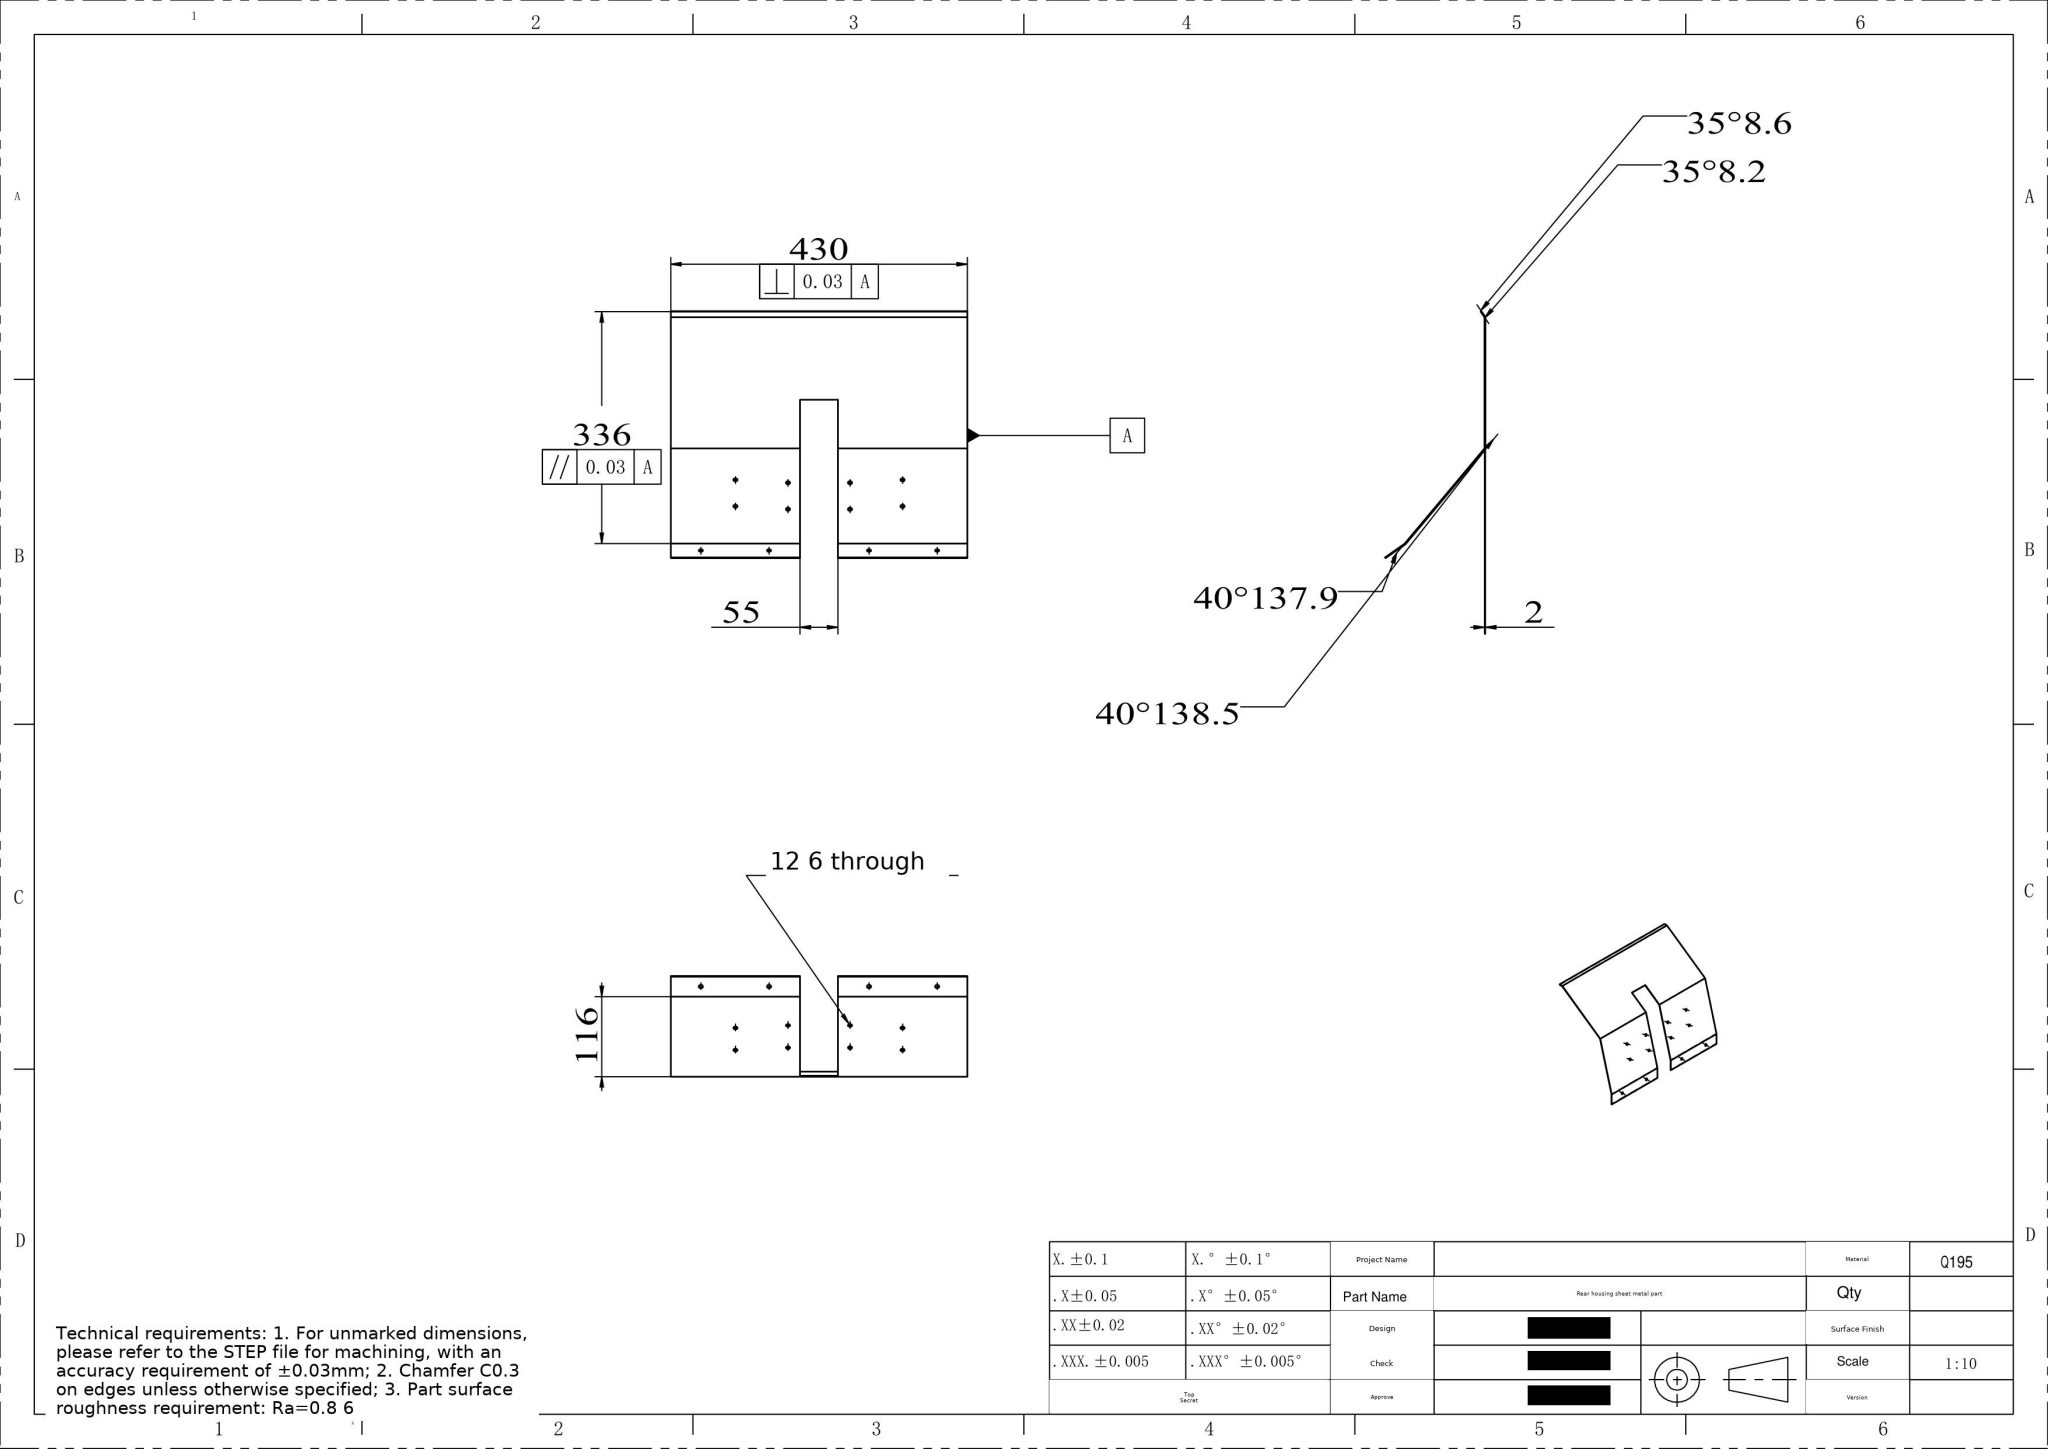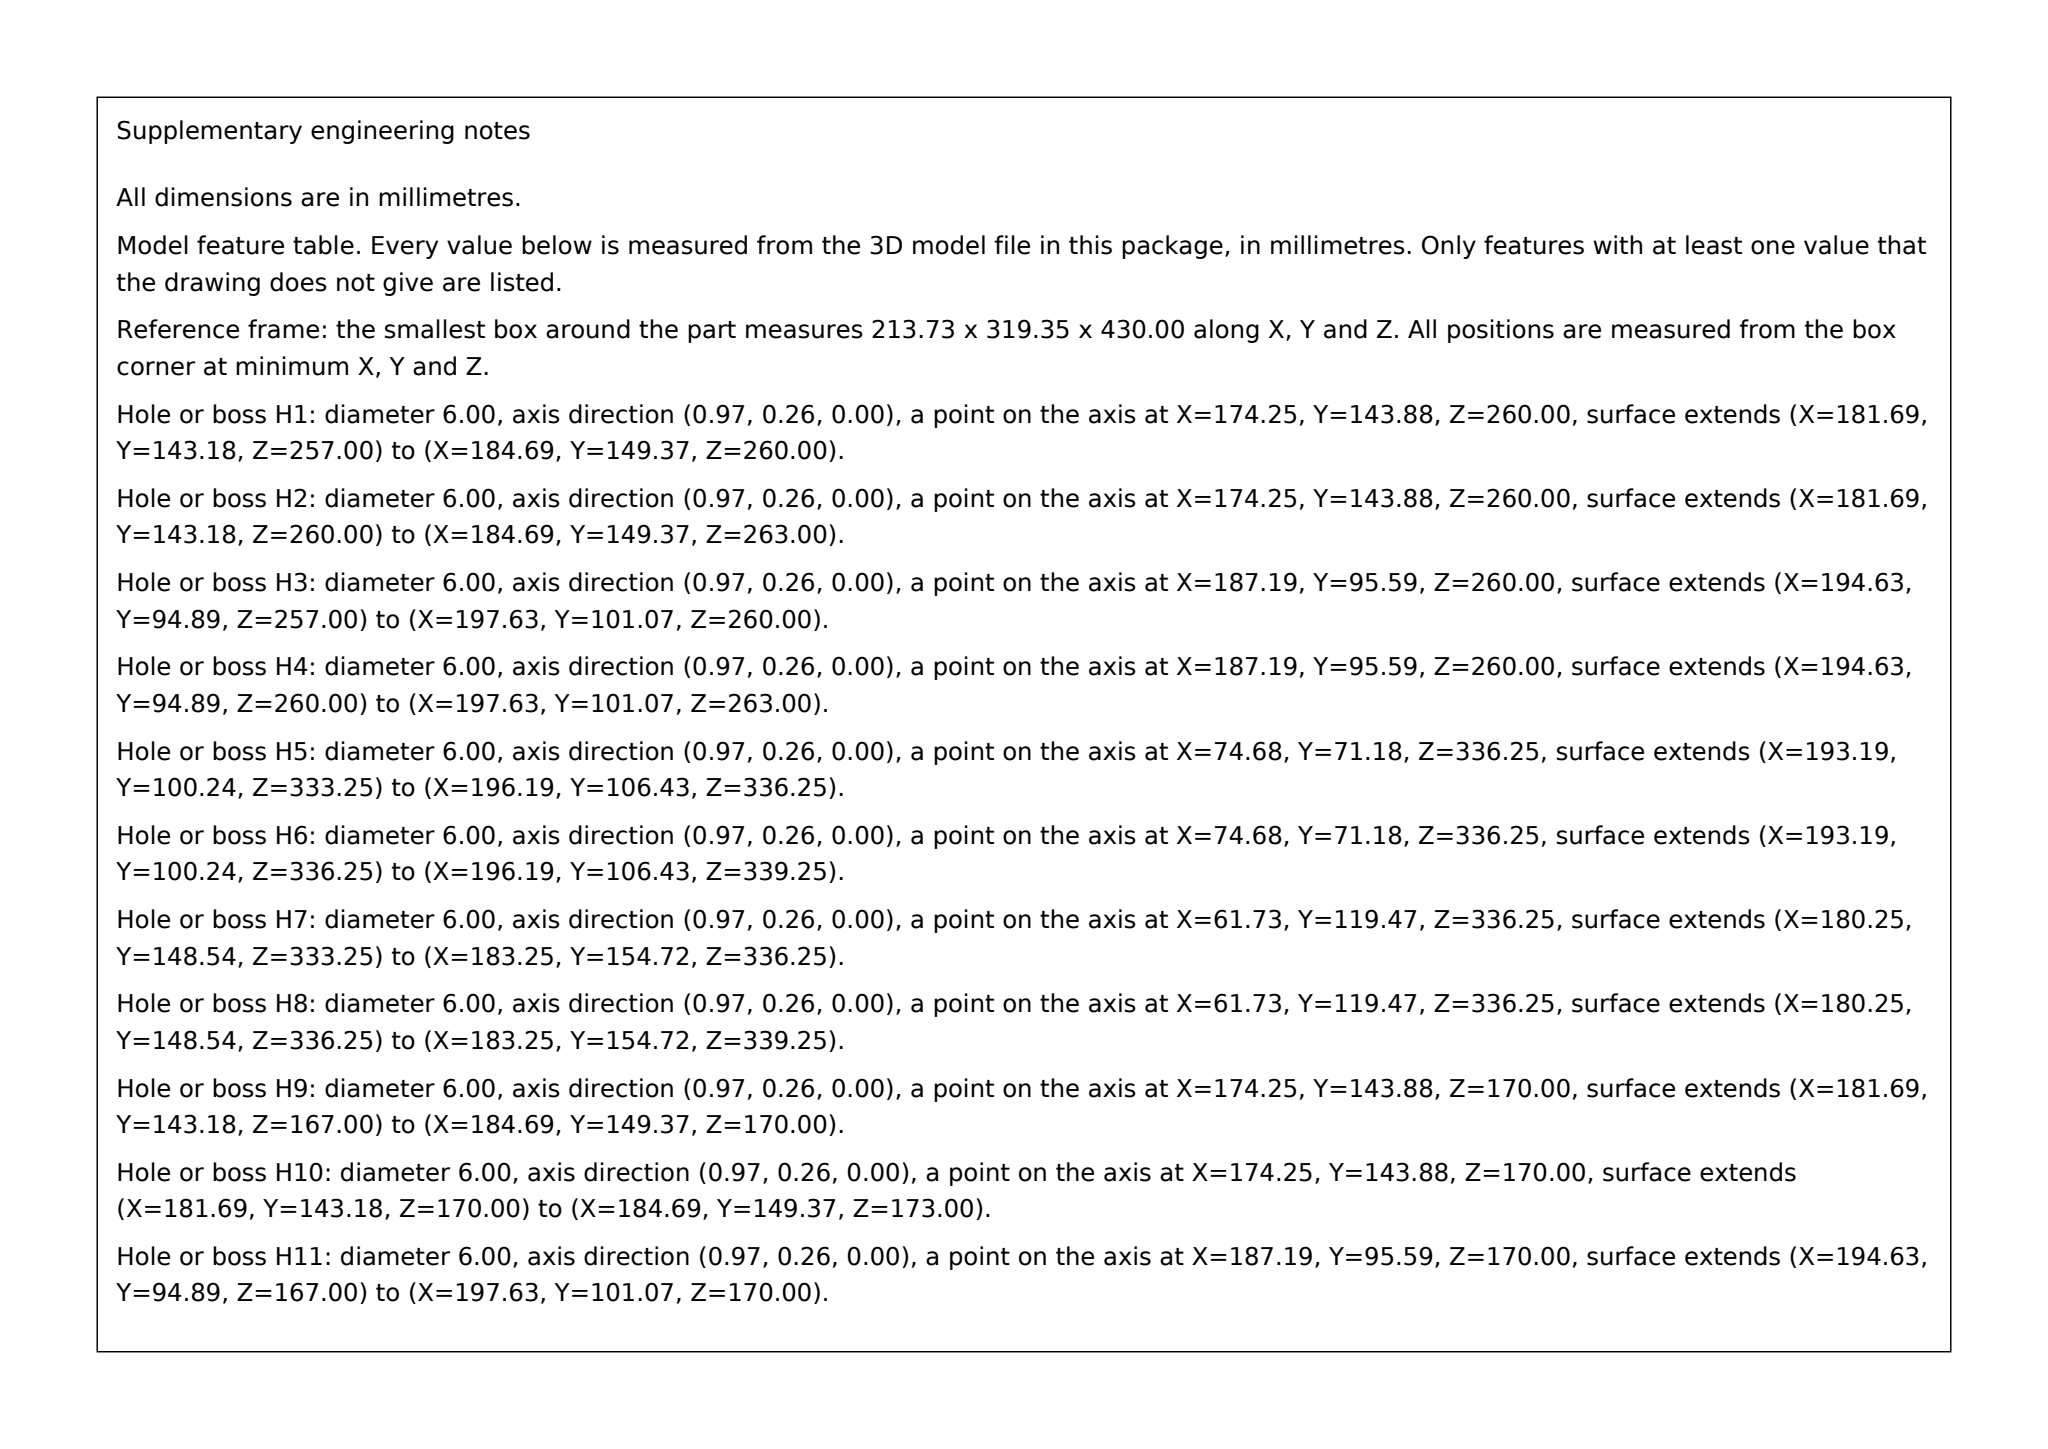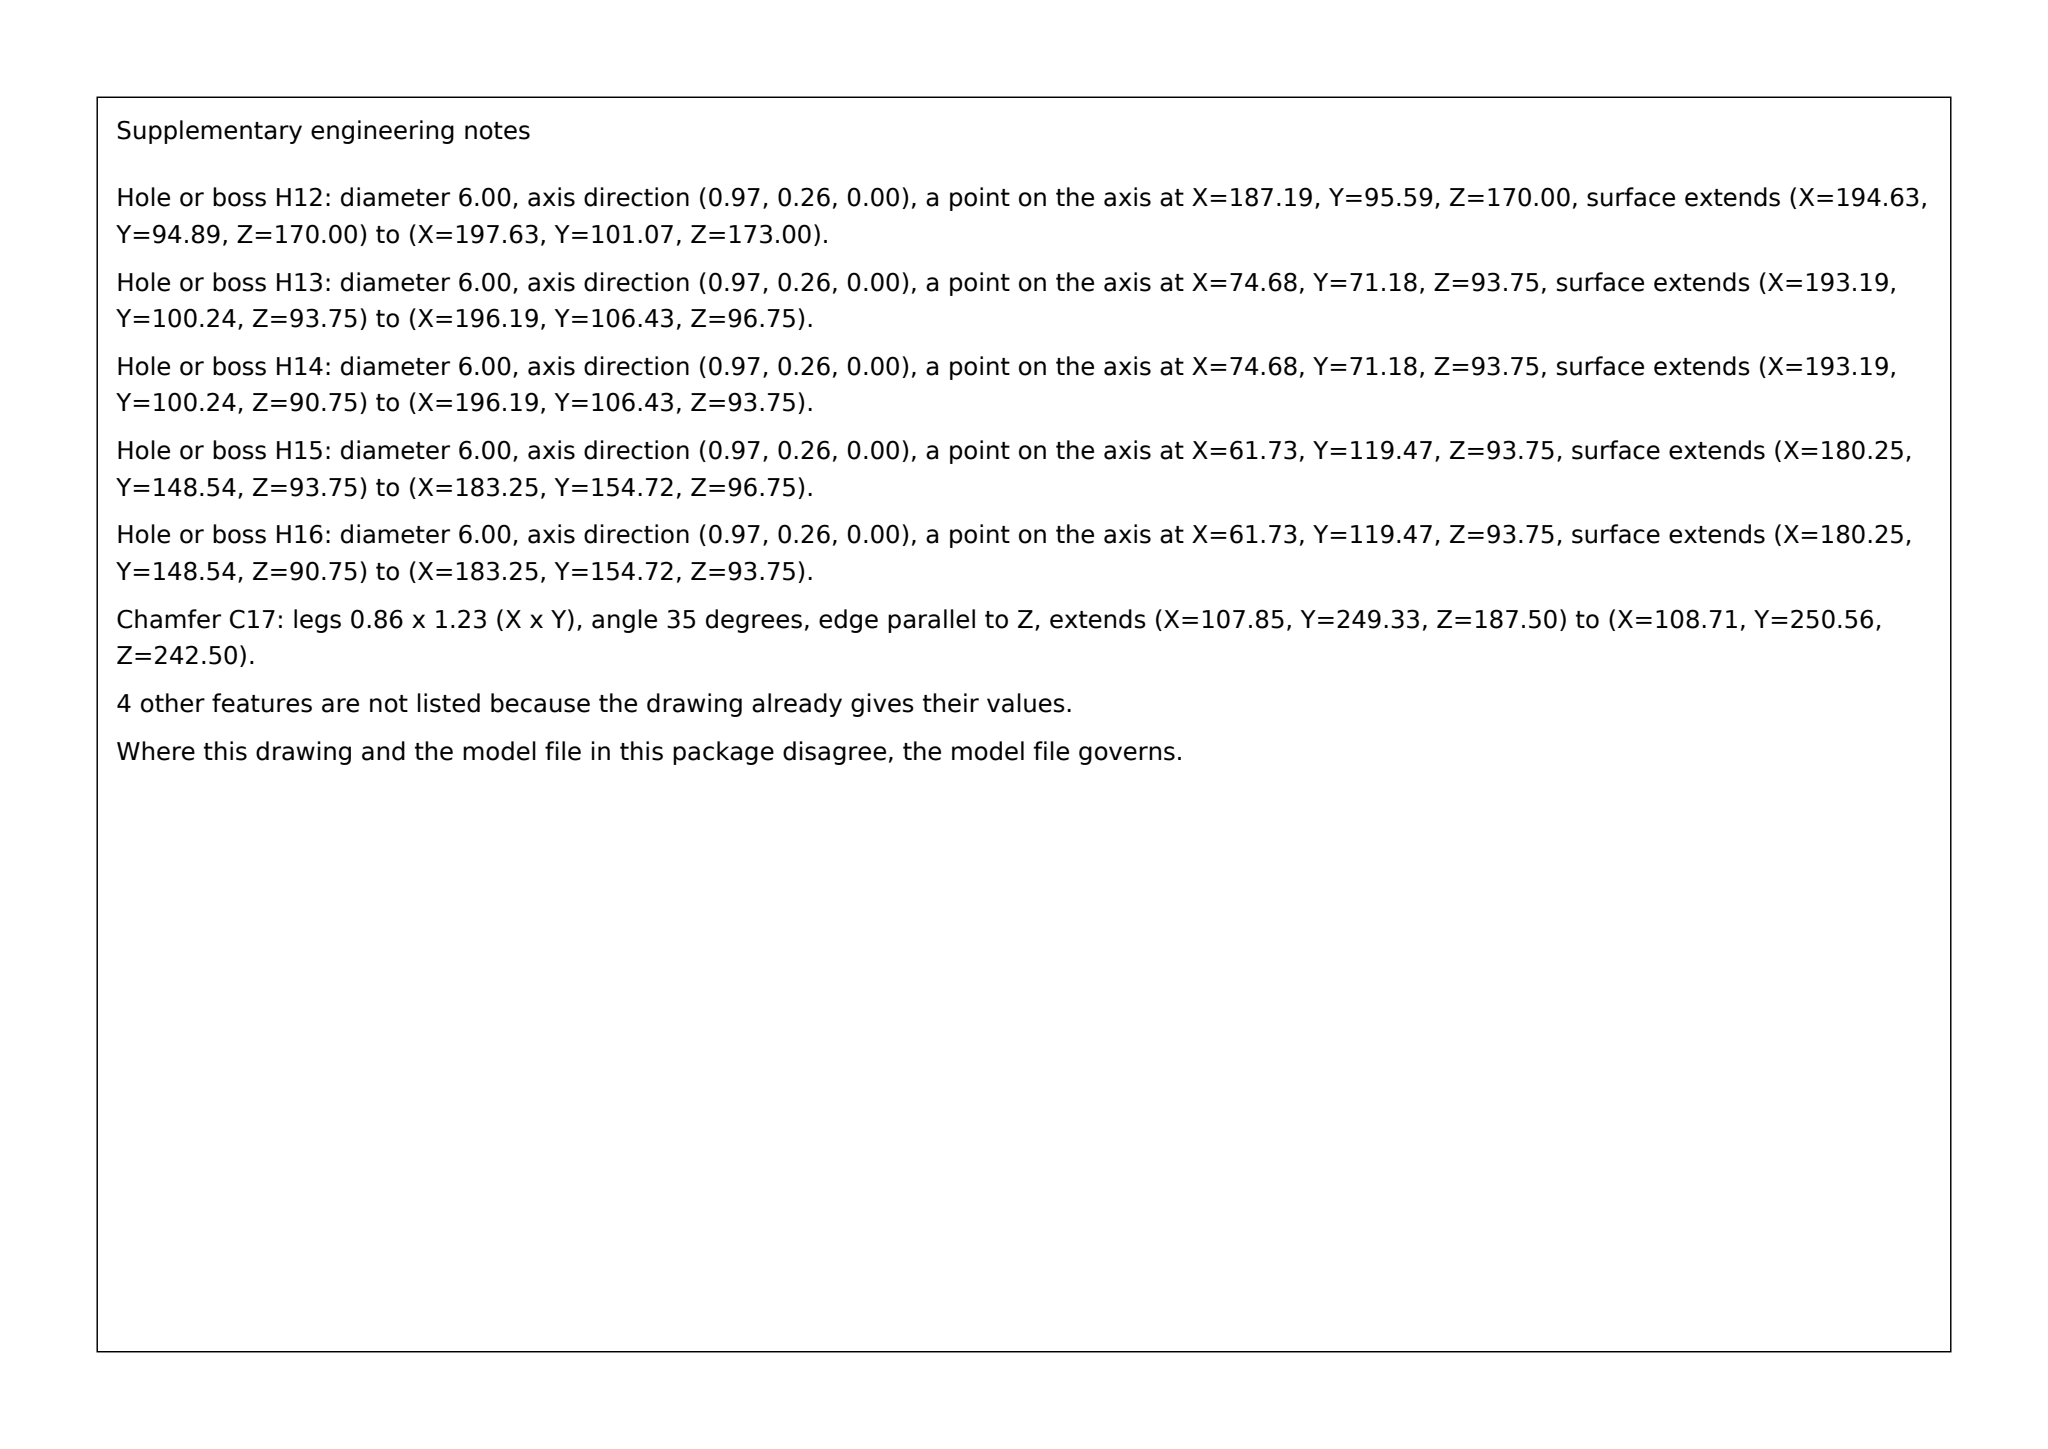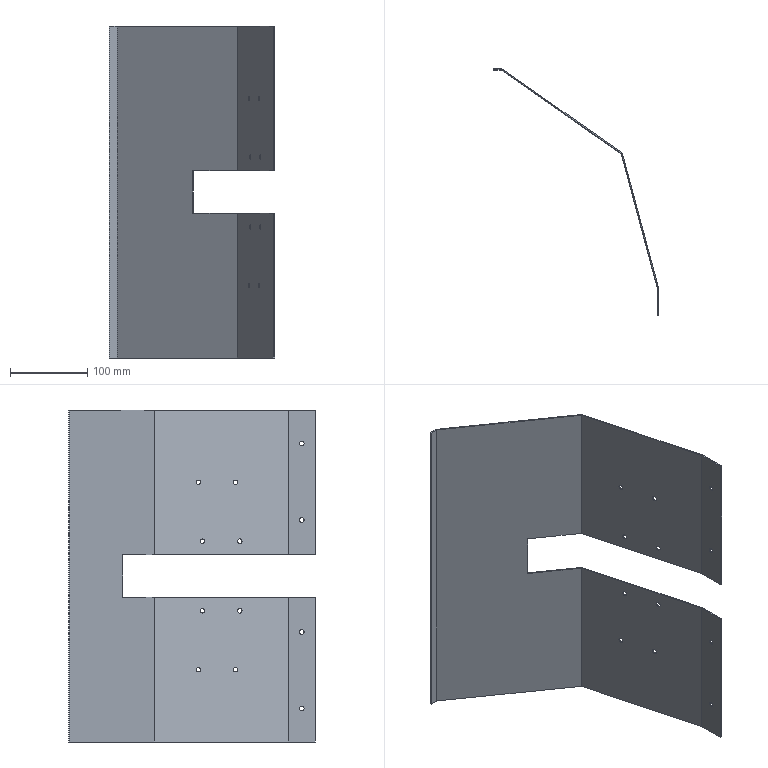Part | SolidWorks | mm | material Q195 | 1 solid | 44 faces | box 213.73 x 319.35 x 430 mm | volume 244331 mm3 | cylinder 24 | plane 20 | commonest cylinder face diameters 6 x24